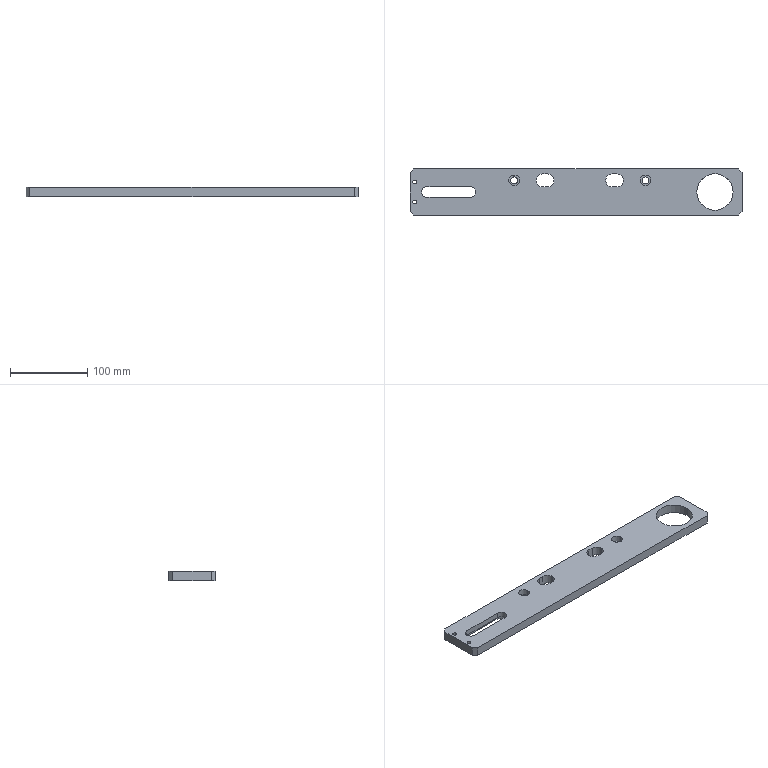Component | SolidWorks | -UpperSlidingSleeveConnectingPlate02-1-1 | 1 solid | 47 faces | volume 263106 mm3 | cylinder 26 | plane 21 | commonest cylinder face diameters 14 x7 17 x6 5 x4 9 x4 20 x3 47 x2